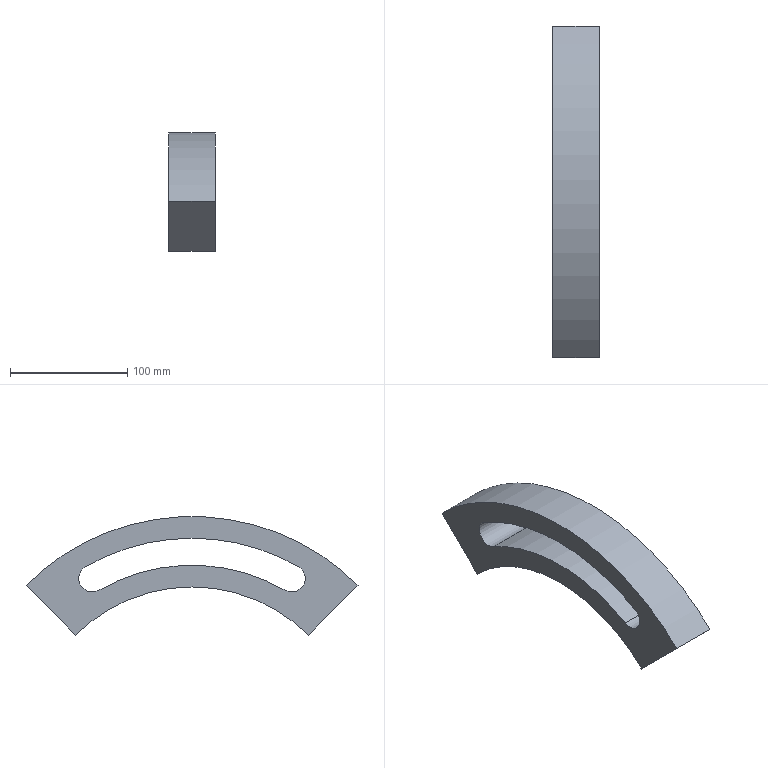Component | NX | BALANCE_BLOCK | 1 solid | 10 faces | box 40 x 282.84 x 101.01 mm | volume 460484 mm3 | cylinder 6 | plane 4 | commonest cylinder face diameters 23 x2 363 x1 280 x1 400 x1 317 x1
STEP:
#1=CARTESIAN_POINT('',(0.,0.,0.));
#2=DIRECTION('',(0.,0.,1.));
#3=DIRECTION('',(1.,0.,0.));
#4=AXIS2_PLACEMENT_3D('',#1,#2,#3);
#5=CARTESIAN_POINT('',(90.,-79.25,137.265));
#6=VERTEX_POINT('',#5);
#7=CARTESIAN_POINT('',(50.,-79.25,137.265));
#8=VERTEX_POINT('',#7);
#9=CARTESIAN_POINT('',(90.,-79.25,137.265));
#10=DIRECTION('',(-1.,0.,0.));
#11=VECTOR('',#10,1.);
#12=LINE('',#9,#11);
#13=CARTESIAN_POINT('',(90.,-85.,147.224));
#14=DIRECTION('',(-1.,0.,0.));
#15=DIRECTION('',(0.,0.,1.));
#16=AXIS2_PLACEMENT_3D('',#13,#14,#15);
#17=CYLINDRICAL_SURFACE('',#16,11.5);
#18=CARTESIAN_POINT('',(2.618,0.));
#19=DIRECTION('',(0.,1.));
#20=VECTOR('',#19,1.);
#21=LINE('',#18,#20);
#22=(GEOMETRIC_REPRESENTATION_CONTEXT(2)PARAMETRIC_REPRESENTATION_CONTEXT()REPRESENTATION_CONTEXT('',''));
#23=DEFINITIONAL_REPRESENTATION('',(#21),#22);
#24=PCURVE('',#17,#23);
#25=CARTESIAN_POINT('',(90.,0.,0.));
#26=DIRECTION('',(-1.,0.,0.));
#27=DIRECTION('',(0.,0.,1.));
#28=AXIS2_PLACEMENT_3D('',#25,#26,#27);
#29=CYLINDRICAL_SURFACE('',#28,158.5);
#30=CARTESIAN_POINT('',(-0.5236,0.));
#31=DIRECTION('',(0.,1.));
#32=VECTOR('',#31,1.);
#33=LINE('',#30,#32);
#34=(GEOMETRIC_REPRESENTATION_CONTEXT(2)PARAMETRIC_REPRESENTATION_CONTEXT()REPRESENTATION_CONTEXT('',''));
#35=DEFINITIONAL_REPRESENTATION('',(#33),#34);
#36=PCURVE('',#29,#35);
#37=SURFACE_CURVE('',#12,(#24,#36),.PCURVE_S1.);
#38=EDGE_CURVE('',#6,#8,#37,.T.);
#39=ORIENTED_EDGE('',*,*,#38,.F.);
#40=CARTESIAN_POINT('',(90.,-90.75,157.184));
#41=VERTEX_POINT('',#40);
#42=CARTESIAN_POINT('',(90.,-85.,147.224));
#43=DIRECTION('',(-1.,0.,0.));
#44=DIRECTION('',(0.,1.,0.));
#45=AXIS2_PLACEMENT_3D('',#42,#43,#44);
#46=CIRCLE('',#45,11.5);
#47=CARTESIAN_POINT('',(1.571,0.));
#48=DIRECTION('',(1.,0.));
#49=VECTOR('',#48,1.);
#50=LINE('',#47,#49);
#51=(GEOMETRIC_REPRESENTATION_CONTEXT(2)PARAMETRIC_REPRESENTATION_CONTEXT()REPRESENTATION_CONTEXT('',''));
#52=DEFINITIONAL_REPRESENTATION('',(#50),#51);
#53=PCURVE('',#17,#52);
#54=CARTESIAN_POINT('',(90.,0.,0.));
#55=DIRECTION('',(-1.,0.,0.));
#56=DIRECTION('',(0.,0.,1.));
#57=AXIS2_PLACEMENT_3D('',#54,#55,#56);
#58=PLANE('',#57);
#59=CARTESIAN_POINT('',(147.224,-85.));
#60=DIRECTION('',(0.,1.));
#61=AXIS2_PLACEMENT_2D('',#59,#60);
#62=CIRCLE('',#61,11.5);
#63=(GEOMETRIC_REPRESENTATION_CONTEXT(2)PARAMETRIC_REPRESENTATION_CONTEXT()REPRESENTATION_CONTEXT('',''));
#64=DEFINITIONAL_REPRESENTATION('',(#62),#63);
#65=PCURVE('',#58,#64);
#66=SURFACE_CURVE('',#46,(#53,#65),.PCURVE_S1.);
#67=EDGE_CURVE('',#6,#41,#66,.T.);
#68=ORIENTED_EDGE('',*,*,#67,.T.);
#69=CARTESIAN_POINT('',(50.,-90.75,157.184));
#70=VERTEX_POINT('',#69);
#71=CARTESIAN_POINT('',(90.,-90.75,157.184));
#72=DIRECTION('',(-1.,0.,0.));
#73=VECTOR('',#72,1.);
#74=LINE('',#71,#73);
#75=CARTESIAN_POINT('',(5.76,0.));
#76=DIRECTION('',(0.,1.));
#77=VECTOR('',#76,1.);
#78=LINE('',#75,#77);
#79=(GEOMETRIC_REPRESENTATION_CONTEXT(2)PARAMETRIC_REPRESENTATION_CONTEXT()REPRESENTATION_CONTEXT('',''));
#80=DEFINITIONAL_REPRESENTATION('',(#78),#79);
#81=PCURVE('',#17,#80);
#82=CARTESIAN_POINT('',(90.,0.,0.));
#83=DIRECTION('',(-1.,0.,0.));
#84=DIRECTION('',(0.,0.,1.));
#85=AXIS2_PLACEMENT_3D('',#82,#83,#84);
#86=CYLINDRICAL_SURFACE('',#85,181.5);
#87=CARTESIAN_POINT('',(5.76,0.));
#88=DIRECTION('',(0.,1.));
#89=VECTOR('',#88,1.);
#90=LINE('',#87,#89);
#91=(GEOMETRIC_REPRESENTATION_CONTEXT(2)PARAMETRIC_REPRESENTATION_CONTEXT()REPRESENTATION_CONTEXT('',''));
#92=DEFINITIONAL_REPRESENTATION('',(#90),#91);
#93=PCURVE('',#86,#92);
#94=SURFACE_CURVE('',#74,(#81,#93),.PCURVE_S1.);
#95=EDGE_CURVE('',#41,#70,#94,.T.);
#96=ORIENTED_EDGE('',*,*,#95,.T.);
#97=CARTESIAN_POINT('',(50.,-85.,147.224));
#98=DIRECTION('',(-1.,0.,0.));
#99=DIRECTION('',(0.,1.,0.));
#100=AXIS2_PLACEMENT_3D('',#97,#98,#99);
#101=CIRCLE('',#100,11.5);
#102=CARTESIAN_POINT('',(1.571,40.));
#103=DIRECTION('',(1.,0.));
#104=VECTOR('',#103,1.);
#105=LINE('',#102,#104);
#106=(GEOMETRIC_REPRESENTATION_CONTEXT(2)PARAMETRIC_REPRESENTATION_CONTEXT()REPRESENTATION_CONTEXT('',''));
#107=DEFINITIONAL_REPRESENTATION('',(#105),#106);
#108=PCURVE('',#17,#107);
#109=CARTESIAN_POINT('',(50.,0.,0.));
#110=DIRECTION('',(-1.,0.,0.));
#111=DIRECTION('',(0.,0.,1.));
#112=AXIS2_PLACEMENT_3D('',#109,#110,#111);
#113=PLANE('',#112);
#114=CARTESIAN_POINT('',(147.224,-85.));
#115=DIRECTION('',(0.,1.));
#116=AXIS2_PLACEMENT_2D('',#114,#115);
#117=CIRCLE('',#116,11.5);
#118=(GEOMETRIC_REPRESENTATION_CONTEXT(2)PARAMETRIC_REPRESENTATION_CONTEXT()REPRESENTATION_CONTEXT('',''));
#119=DEFINITIONAL_REPRESENTATION('',(#117),#118);
#120=PCURVE('',#113,#119);
#121=SURFACE_CURVE('',#101,(#108,#120),.PCURVE_S1.);
#122=EDGE_CURVE('',#8,#70,#121,.T.);
#123=ORIENTED_EDGE('',*,*,#122,.F.);
#124=EDGE_LOOP('',(#39,#68,#96,#123));
#125=FACE_BOUND('',#124,.F.);
#126=ADVANCED_FACE('',(#125),#17,.F.);
#127=ORIENTED_EDGE('',*,*,#95,.F.);
#128=CARTESIAN_POINT('',(90.,90.75,157.184));
#129=VERTEX_POINT('',#128);
#130=CARTESIAN_POINT('',(90.,0.,0.));
#131=DIRECTION('',(-1.,0.,0.));
#132=DIRECTION('',(0.,1.,0.));
#133=AXIS2_PLACEMENT_3D('',#130,#131,#132);
#134=CIRCLE('',#133,181.5);
#135=CARTESIAN_POINT('',(1.571,0.));
#136=DIRECTION('',(1.,0.));
#137=VECTOR('',#136,1.);
#138=LINE('',#135,#137);
#139=(GEOMETRIC_REPRESENTATION_CONTEXT(2)PARAMETRIC_REPRESENTATION_CONTEXT()REPRESENTATION_CONTEXT('',''));
#140=DEFINITIONAL_REPRESENTATION('',(#138),#139);
#141=PCURVE('',#86,#140);
#142=CARTESIAN_POINT('',(0.,0.));
#143=DIRECTION('',(0.,1.));
#144=AXIS2_PLACEMENT_2D('',#142,#143);
#145=CIRCLE('',#144,181.5);
#146=(GEOMETRIC_REPRESENTATION_CONTEXT(2)PARAMETRIC_REPRESENTATION_CONTEXT()REPRESENTATION_CONTEXT('',''));
#147=DEFINITIONAL_REPRESENTATION('',(#145),#146);
#148=PCURVE('',#58,#147);
#149=SURFACE_CURVE('',#134,(#141,#148),.PCURVE_S1.);
#150=EDGE_CURVE('',#41,#129,#149,.T.);
#151=ORIENTED_EDGE('',*,*,#150,.T.);
#152=CARTESIAN_POINT('',(50.,90.75,157.184));
#153=VERTEX_POINT('',#152);
#154=CARTESIAN_POINT('',(90.,90.75,157.184));
#155=DIRECTION('',(-1.,0.,0.));
#156=VECTOR('',#155,1.);
#157=LINE('',#154,#156);
#158=CARTESIAN_POINT('',(6.807,0.));
#159=DIRECTION('',(0.,1.));
#160=VECTOR('',#159,1.);
#161=LINE('',#158,#160);
#162=(GEOMETRIC_REPRESENTATION_CONTEXT(2)PARAMETRIC_REPRESENTATION_CONTEXT()REPRESENTATION_CONTEXT('',''));
#163=DEFINITIONAL_REPRESENTATION('',(#161),#162);
#164=PCURVE('',#86,#163);
#165=CARTESIAN_POINT('',(90.,85.,147.224));
#166=DIRECTION('',(-1.,0.,0.));
#167=DIRECTION('',(0.,0.,1.));
#168=AXIS2_PLACEMENT_3D('',#165,#166,#167);
#169=CYLINDRICAL_SURFACE('',#168,11.5);
#170=CARTESIAN_POINT('',(0.5236,0.));
#171=DIRECTION('',(0.,1.));
#172=VECTOR('',#171,1.);
#173=LINE('',#170,#172);
#174=(GEOMETRIC_REPRESENTATION_CONTEXT(2)PARAMETRIC_REPRESENTATION_CONTEXT()REPRESENTATION_CONTEXT('',''));
#175=DEFINITIONAL_REPRESENTATION('',(#173),#174);
#176=PCURVE('',#169,#175);
#177=SURFACE_CURVE('',#157,(#164,#176),.PCURVE_S1.);
#178=EDGE_CURVE('',#129,#153,#177,.T.);
#179=ORIENTED_EDGE('',*,*,#178,.T.);
#180=CARTESIAN_POINT('',(50.,0.,0.));
#181=DIRECTION('',(-1.,0.,0.));
#182=DIRECTION('',(0.,1.,0.));
#183=AXIS2_PLACEMENT_3D('',#180,#181,#182);
#184=CIRCLE('',#183,181.5);
#185=CARTESIAN_POINT('',(1.571,40.));
#186=DIRECTION('',(1.,0.));
#187=VECTOR('',#186,1.);
#188=LINE('',#185,#187);
#189=(GEOMETRIC_REPRESENTATION_CONTEXT(2)PARAMETRIC_REPRESENTATION_CONTEXT()REPRESENTATION_CONTEXT('',''));
#190=DEFINITIONAL_REPRESENTATION('',(#188),#189);
#191=PCURVE('',#86,#190);
#192=CARTESIAN_POINT('',(0.,0.));
#193=DIRECTION('',(0.,1.));
#194=AXIS2_PLACEMENT_2D('',#192,#193);
#195=CIRCLE('',#194,181.5);
#196=(GEOMETRIC_REPRESENTATION_CONTEXT(2)PARAMETRIC_REPRESENTATION_CONTEXT()REPRESENTATION_CONTEXT('',''));
#197=DEFINITIONAL_REPRESENTATION('',(#195),#196);
#198=PCURVE('',#113,#197);
#199=SURFACE_CURVE('',#184,(#191,#198),.PCURVE_S1.);
#200=EDGE_CURVE('',#70,#153,#199,.T.);
#201=ORIENTED_EDGE('',*,*,#200,.F.);
#202=EDGE_LOOP('',(#127,#151,#179,#201));
#203=FACE_BOUND('',#202,.F.);
#204=ADVANCED_FACE('',(#203),#86,.F.);
#205=ORIENTED_EDGE('',*,*,#178,.F.);
#206=CARTESIAN_POINT('',(90.,79.25,137.265));
#207=VERTEX_POINT('',#206);
#208=CARTESIAN_POINT('',(90.,85.,147.224));
#209=DIRECTION('',(-1.,0.,0.));
#210=DIRECTION('',(0.,1.,0.));
#211=AXIS2_PLACEMENT_3D('',#208,#209,#210);
#212=CIRCLE('',#211,11.5);
#213=CARTESIAN_POINT('',(-4.712,0.));
#214=DIRECTION('',(1.,0.));
#215=VECTOR('',#214,1.);
#216=LINE('',#213,#215);
#217=(GEOMETRIC_REPRESENTATION_CONTEXT(2)PARAMETRIC_REPRESENTATION_CONTEXT()REPRESENTATION_CONTEXT('',''));
#218=DEFINITIONAL_REPRESENTATION('',(#216),#217);
#219=PCURVE('',#169,#218);
#220=CARTESIAN_POINT('',(147.224,85.));
#221=DIRECTION('',(0.,1.));
#222=AXIS2_PLACEMENT_2D('',#220,#221);
#223=CIRCLE('',#222,11.5);
#224=(GEOMETRIC_REPRESENTATION_CONTEXT(2)PARAMETRIC_REPRESENTATION_CONTEXT()REPRESENTATION_CONTEXT('',''));
#225=DEFINITIONAL_REPRESENTATION('',(#223),#224);
#226=PCURVE('',#58,#225);
#227=SURFACE_CURVE('',#212,(#219,#226),.PCURVE_S1.);
#228=EDGE_CURVE('',#129,#207,#227,.T.);
#229=ORIENTED_EDGE('',*,*,#228,.T.);
#230=CARTESIAN_POINT('',(50.,79.25,137.265));
#231=VERTEX_POINT('',#230);
#232=CARTESIAN_POINT('',(90.,79.25,137.265));
#233=DIRECTION('',(-1.,0.,0.));
#234=VECTOR('',#233,1.);
#235=LINE('',#232,#234);
#236=CARTESIAN_POINT('',(3.665,0.));
#237=DIRECTION('',(0.,1.));
#238=VECTOR('',#237,1.);
#239=LINE('',#236,#238);
#240=(GEOMETRIC_REPRESENTATION_CONTEXT(2)PARAMETRIC_REPRESENTATION_CONTEXT()REPRESENTATION_CONTEXT('',''));
#241=DEFINITIONAL_REPRESENTATION('',(#239),#240);
#242=PCURVE('',#169,#241);
#243=CARTESIAN_POINT('',(0.5236,0.));
#244=DIRECTION('',(0.,1.));
#245=VECTOR('',#244,1.);
#246=LINE('',#243,#245);
#247=(GEOMETRIC_REPRESENTATION_CONTEXT(2)PARAMETRIC_REPRESENTATION_CONTEXT()REPRESENTATION_CONTEXT('',''));
#248=DEFINITIONAL_REPRESENTATION('',(#246),#247);
#249=PCURVE('',#29,#248);
#250=SURFACE_CURVE('',#235,(#242,#249),.PCURVE_S1.);
#251=EDGE_CURVE('',#207,#231,#250,.T.);
#252=ORIENTED_EDGE('',*,*,#251,.T.);
#253=CARTESIAN_POINT('',(50.,85.,147.224));
#254=DIRECTION('',(-1.,0.,0.));
#255=DIRECTION('',(0.,1.,0.));
#256=AXIS2_PLACEMENT_3D('',#253,#254,#255);
#257=CIRCLE('',#256,11.5);
#258=CARTESIAN_POINT('',(-4.712,40.));
#259=DIRECTION('',(1.,0.));
#260=VECTOR('',#259,1.);
#261=LINE('',#258,#260);
#262=(GEOMETRIC_REPRESENTATION_CONTEXT(2)PARAMETRIC_REPRESENTATION_CONTEXT()REPRESENTATION_CONTEXT('',''));
#263=DEFINITIONAL_REPRESENTATION('',(#261),#262);
#264=PCURVE('',#169,#263);
#265=CARTESIAN_POINT('',(147.224,85.));
#266=DIRECTION('',(0.,1.));
#267=AXIS2_PLACEMENT_2D('',#265,#266);
#268=CIRCLE('',#267,11.5);
#269=(GEOMETRIC_REPRESENTATION_CONTEXT(2)PARAMETRIC_REPRESENTATION_CONTEXT()REPRESENTATION_CONTEXT('',''));
#270=DEFINITIONAL_REPRESENTATION('',(#268),#269);
#271=PCURVE('',#113,#270);
#272=SURFACE_CURVE('',#257,(#264,#271),.PCURVE_S1.);
#273=EDGE_CURVE('',#153,#231,#272,.T.);
#274=ORIENTED_EDGE('',*,*,#273,.F.);
#275=EDGE_LOOP('',(#205,#229,#252,#274));
#276=FACE_BOUND('',#275,.F.);
#277=ADVANCED_FACE('',(#276),#169,.F.);
#278=CARTESIAN_POINT('',(50.,-141.421,141.421));
#279=VERTEX_POINT('',#278);
#280=CARTESIAN_POINT('',(50.,-98.995,98.995));
#281=VERTEX_POINT('',#280);
#282=CARTESIAN_POINT('',(50.,-141.421,141.421));
#283=DIRECTION('',(0.,0.7071,-0.7071));
#284=VECTOR('',#283,1.);
#285=LINE('',#282,#284);
#286=CARTESIAN_POINT('',(90.,-141.421,141.421));
#287=DIRECTION('',(0.,0.7071,0.7071));
#288=DIRECTION('',(0.,-0.7071,0.7071));
#289=AXIS2_PLACEMENT_3D('',#286,#287,#288);
#290=PLANE('',#289);
#291=CARTESIAN_POINT('',(0.,-40.));
#292=DIRECTION('',(-1.,0.));
#293=VECTOR('',#292,1.);
#294=LINE('',#291,#293);
#295=(GEOMETRIC_REPRESENTATION_CONTEXT(2)PARAMETRIC_REPRESENTATION_CONTEXT()REPRESENTATION_CONTEXT('',''));
#296=DEFINITIONAL_REPRESENTATION('',(#294),#295);
#297=PCURVE('',#290,#296);
#298=CARTESIAN_POINT('',(141.421,-141.421));
#299=DIRECTION('',(-0.7071,0.7071));
#300=VECTOR('',#299,1.);
#301=LINE('',#298,#300);
#302=(GEOMETRIC_REPRESENTATION_CONTEXT(2)PARAMETRIC_REPRESENTATION_CONTEXT()REPRESENTATION_CONTEXT('',''));
#303=DEFINITIONAL_REPRESENTATION('',(#301),#302);
#304=PCURVE('',#113,#303);
#305=SURFACE_CURVE('',#285,(#297,#304),.PCURVE_S1.);
#306=EDGE_CURVE('',#279,#281,#305,.T.);
#307=ORIENTED_EDGE('',*,*,#306,.T.);
#308=CARTESIAN_POINT('',(90.,-98.995,98.995));
#309=VERTEX_POINT('',#308);
#310=CARTESIAN_POINT('',(90.,-98.995,98.995));
#311=DIRECTION('',(-1.,0.,0.));
#312=VECTOR('',#311,1.);
#313=LINE('',#310,#312);
#314=CARTESIAN_POINT('',(-60.,0.));
#315=DIRECTION('',(0.,-1.));
#316=VECTOR('',#315,1.);
#317=LINE('',#314,#316);
#318=(GEOMETRIC_REPRESENTATION_CONTEXT(2)PARAMETRIC_REPRESENTATION_CONTEXT()REPRESENTATION_CONTEXT('',''));
#319=DEFINITIONAL_REPRESENTATION('',(#317),#318);
#320=PCURVE('',#290,#319);
#321=CARTESIAN_POINT('',(90.,0.,0.));
#322=DIRECTION('',(-1.,0.,0.));
#323=DIRECTION('',(0.,0.,1.));
#324=AXIS2_PLACEMENT_3D('',#321,#322,#323);
#325=CYLINDRICAL_SURFACE('',#324,140.);
#326=CARTESIAN_POINT('',(5.498,0.));
#327=DIRECTION('',(0.,1.));
#328=VECTOR('',#327,1.);
#329=LINE('',#326,#328);
#330=(GEOMETRIC_REPRESENTATION_CONTEXT(2)PARAMETRIC_REPRESENTATION_CONTEXT()REPRESENTATION_CONTEXT('',''));
#331=DEFINITIONAL_REPRESENTATION('',(#329),#330);
#332=PCURVE('',#325,#331);
#333=SURFACE_CURVE('',#313,(#320,#332),.PCURVE_S1.);
#334=EDGE_CURVE('',#309,#281,#333,.T.);
#335=ORIENTED_EDGE('',*,*,#334,.F.);
#336=CARTESIAN_POINT('',(90.,-141.421,141.421));
#337=VERTEX_POINT('',#336);
#338=CARTESIAN_POINT('',(90.,-141.421,141.421));
#339=DIRECTION('',(0.,0.7071,-0.7071));
#340=VECTOR('',#339,1.);
#341=LINE('',#338,#340);
#342=CARTESIAN_POINT('',(0.,0.));
#343=DIRECTION('',(-1.,0.));
#344=VECTOR('',#343,1.);
#345=LINE('',#342,#344);
#346=(GEOMETRIC_REPRESENTATION_CONTEXT(2)PARAMETRIC_REPRESENTATION_CONTEXT()REPRESENTATION_CONTEXT('',''));
#347=DEFINITIONAL_REPRESENTATION('',(#345),#346);
#348=PCURVE('',#290,#347);
#349=CARTESIAN_POINT('',(141.421,-141.421));
#350=DIRECTION('',(-0.7071,0.7071));
#351=VECTOR('',#350,1.);
#352=LINE('',#349,#351);
#353=(GEOMETRIC_REPRESENTATION_CONTEXT(2)PARAMETRIC_REPRESENTATION_CONTEXT()REPRESENTATION_CONTEXT('',''));
#354=DEFINITIONAL_REPRESENTATION('',(#352),#353);
#355=PCURVE('',#58,#354);
#356=SURFACE_CURVE('',#341,(#348,#355),.PCURVE_S1.);
#357=EDGE_CURVE('',#337,#309,#356,.T.);
#358=ORIENTED_EDGE('',*,*,#357,.F.);
#359=CARTESIAN_POINT('',(90.,-141.421,141.421));
#360=DIRECTION('',(-1.,0.,0.));
#361=VECTOR('',#360,1.);
#362=LINE('',#359,#361);
#363=CARTESIAN_POINT('',(0.,0.));
#364=DIRECTION('',(0.,-1.));
#365=VECTOR('',#364,1.);
#366=LINE('',#363,#365);
#367=(GEOMETRIC_REPRESENTATION_CONTEXT(2)PARAMETRIC_REPRESENTATION_CONTEXT()REPRESENTATION_CONTEXT('',''));
#368=DEFINITIONAL_REPRESENTATION('',(#366),#367);
#369=PCURVE('',#290,#368);
#370=CARTESIAN_POINT('',(90.,0.,0.));
#371=DIRECTION('',(-1.,0.,0.));
#372=DIRECTION('',(0.,0.,1.));
#373=AXIS2_PLACEMENT_3D('',#370,#371,#372);
#374=CYLINDRICAL_SURFACE('',#373,200.);
#375=CARTESIAN_POINT('',(-0.7854,0.));
#376=DIRECTION('',(0.,1.));
#377=VECTOR('',#376,1.);
#378=LINE('',#375,#377);
#379=(GEOMETRIC_REPRESENTATION_CONTEXT(2)PARAMETRIC_REPRESENTATION_CONTEXT()REPRESENTATION_CONTEXT('',''));
#380=DEFINITIONAL_REPRESENTATION('',(#378),#379);
#381=PCURVE('',#374,#380);
#382=SURFACE_CURVE('',#362,(#369,#381),.PCURVE_S1.);
#383=EDGE_CURVE('',#337,#279,#382,.T.);
#384=ORIENTED_EDGE('',*,*,#383,.T.);
#385=EDGE_LOOP('',(#307,#335,#358,#384));
#386=FACE_BOUND('',#385,.T.);
#387=ADVANCED_FACE('',(#386),#290,.F.);
#388=ORIENTED_EDGE('',*,*,#334,.F.);
#389=CARTESIAN_POINT('',(90.,98.995,98.995));
#390=VERTEX_POINT('',#389);
#391=CARTESIAN_POINT('',(90.,0.,0.));
#392=DIRECTION('',(-1.,0.,0.));
#393=DIRECTION('',(0.,1.,0.));
#394=AXIS2_PLACEMENT_3D('',#391,#392,#393);
#395=CIRCLE('',#394,140.);
#396=CARTESIAN_POINT('',(1.571,0.));
#397=DIRECTION('',(1.,0.));
#398=VECTOR('',#397,1.);
#399=LINE('',#396,#398);
#400=(GEOMETRIC_REPRESENTATION_CONTEXT(2)PARAMETRIC_REPRESENTATION_CONTEXT()REPRESENTATION_CONTEXT('',''));
#401=DEFINITIONAL_REPRESENTATION('',(#399),#400);
#402=PCURVE('',#325,#401);
#403=CARTESIAN_POINT('',(0.,0.));
#404=DIRECTION('',(0.,1.));
#405=AXIS2_PLACEMENT_2D('',#403,#404);
#406=CIRCLE('',#405,140.);
#407=(GEOMETRIC_REPRESENTATION_CONTEXT(2)PARAMETRIC_REPRESENTATION_CONTEXT()REPRESENTATION_CONTEXT('',''));
#408=DEFINITIONAL_REPRESENTATION('',(#406),#407);
#409=PCURVE('',#58,#408);
#410=SURFACE_CURVE('',#395,(#402,#409),.PCURVE_S1.);
#411=EDGE_CURVE('',#309,#390,#410,.T.);
#412=ORIENTED_EDGE('',*,*,#411,.T.);
#413=CARTESIAN_POINT('',(50.,98.995,98.995));
#414=VERTEX_POINT('',#413);
#415=CARTESIAN_POINT('',(90.,98.995,98.995));
#416=DIRECTION('',(-1.,0.,0.));
#417=VECTOR('',#416,1.);
#418=LINE('',#415,#417);
#419=CARTESIAN_POINT('',(7.069,0.));
#420=DIRECTION('',(0.,1.));
#421=VECTOR('',#420,1.);
#422=LINE('',#419,#421);
#423=(GEOMETRIC_REPRESENTATION_CONTEXT(2)PARAMETRIC_REPRESENTATION_CONTEXT()REPRESENTATION_CONTEXT('',''));
#424=DEFINITIONAL_REPRESENTATION('',(#422),#423);
#425=PCURVE('',#325,#424);
#426=CARTESIAN_POINT('',(90.,98.995,98.995));
#427=DIRECTION('',(0.,-0.7071,0.7071));
#428=DIRECTION('',(0.,-0.7071,-0.7071));
#429=AXIS2_PLACEMENT_3D('',#426,#427,#428);
#430=PLANE('',#429);
#431=CARTESIAN_POINT('',(0.,0.));
#432=DIRECTION('',(0.,-1.));
#433=VECTOR('',#432,1.);
#434=LINE('',#431,#433);
#435=(GEOMETRIC_REPRESENTATION_CONTEXT(2)PARAMETRIC_REPRESENTATION_CONTEXT()REPRESENTATION_CONTEXT('',''));
#436=DEFINITIONAL_REPRESENTATION('',(#434),#435);
#437=PCURVE('',#430,#436);
#438=SURFACE_CURVE('',#418,(#425,#437),.PCURVE_S1.);
#439=EDGE_CURVE('',#390,#414,#438,.T.);
#440=ORIENTED_EDGE('',*,*,#439,.T.);
#441=CARTESIAN_POINT('',(50.,0.,0.));
#442=DIRECTION('',(-1.,0.,0.));
#443=DIRECTION('',(0.,1.,0.));
#444=AXIS2_PLACEMENT_3D('',#441,#442,#443);
#445=CIRCLE('',#444,140.);
#446=CARTESIAN_POINT('',(1.571,40.));
#447=DIRECTION('',(1.,0.));
#448=VECTOR('',#447,1.);
#449=LINE('',#446,#448);
#450=(GEOMETRIC_REPRESENTATION_CONTEXT(2)PARAMETRIC_REPRESENTATION_CONTEXT()REPRESENTATION_CONTEXT('',''));
#451=DEFINITIONAL_REPRESENTATION('',(#449),#450);
#452=PCURVE('',#325,#451);
#453=CARTESIAN_POINT('',(0.,0.));
#454=DIRECTION('',(0.,1.));
#455=AXIS2_PLACEMENT_2D('',#453,#454);
#456=CIRCLE('',#455,140.);
#457=(GEOMETRIC_REPRESENTATION_CONTEXT(2)PARAMETRIC_REPRESENTATION_CONTEXT()REPRESENTATION_CONTEXT('',''));
#458=DEFINITIONAL_REPRESENTATION('',(#456),#457);
#459=PCURVE('',#113,#458);
#460=SURFACE_CURVE('',#445,(#452,#459),.PCURVE_S1.);
#461=EDGE_CURVE('',#281,#414,#460,.T.);
#462=ORIENTED_EDGE('',*,*,#461,.F.);
#463=EDGE_LOOP('',(#388,#412,#440,#462));
#464=FACE_BOUND('',#463,.F.);
#465=ADVANCED_FACE('',(#464),#325,.F.);
#466=CARTESIAN_POINT('',(50.,141.421,141.421));
#467=VERTEX_POINT('',#466);
#468=CARTESIAN_POINT('',(50.,98.995,98.995));
#469=DIRECTION('',(0.,0.7071,0.7071));
#470=VECTOR('',#469,1.);
#471=LINE('',#468,#470);
#472=CARTESIAN_POINT('',(0.,-40.));
#473=DIRECTION('',(-1.,0.));
#474=VECTOR('',#473,1.);
#475=LINE('',#472,#474);
#476=(GEOMETRIC_REPRESENTATION_CONTEXT(2)PARAMETRIC_REPRESENTATION_CONTEXT()REPRESENTATION_CONTEXT('',''));
#477=DEFINITIONAL_REPRESENTATION('',(#475),#476);
#478=PCURVE('',#430,#477);
#479=CARTESIAN_POINT('',(98.995,98.995));
#480=DIRECTION('',(0.7071,0.7071));
#481=VECTOR('',#480,1.);
#482=LINE('',#479,#481);
#483=(GEOMETRIC_REPRESENTATION_CONTEXT(2)PARAMETRIC_REPRESENTATION_CONTEXT()REPRESENTATION_CONTEXT('',''));
#484=DEFINITIONAL_REPRESENTATION('',(#482),#483);
#485=PCURVE('',#113,#484);
#486=SURFACE_CURVE('',#471,(#478,#485),.PCURVE_S1.);
#487=EDGE_CURVE('',#414,#467,#486,.T.);
#488=ORIENTED_EDGE('',*,*,#487,.T.);
#489=CARTESIAN_POINT('',(90.,141.421,141.421));
#490=VERTEX_POINT('',#489);
#491=CARTESIAN_POINT('',(90.,141.421,141.421));
#492=DIRECTION('',(-1.,0.,0.));
#493=VECTOR('',#492,1.);
#494=LINE('',#491,#493);
#495=CARTESIAN_POINT('',(-60.,0.));
#496=DIRECTION('',(0.,-1.));
#497=VECTOR('',#496,1.);
#498=LINE('',#495,#497);
#499=(GEOMETRIC_REPRESENTATION_CONTEXT(2)PARAMETRIC_REPRESENTATION_CONTEXT()REPRESENTATION_CONTEXT('',''));
#500=DEFINITIONAL_REPRESENTATION('',(#498),#499);
#501=PCURVE('',#430,#500);
#502=CARTESIAN_POINT('',(0.7854,0.));
#503=DIRECTION('',(0.,1.));
#504=VECTOR('',#503,1.);
#505=LINE('',#502,#504);
#506=(GEOMETRIC_REPRESENTATION_CONTEXT(2)PARAMETRIC_REPRESENTATION_CONTEXT()REPRESENTATION_CONTEXT('',''));
#507=DEFINITIONAL_REPRESENTATION('',(#505),#506);
#508=PCURVE('',#374,#507);
#509=SURFACE_CURVE('',#494,(#501,#508),.PCURVE_S1.);
#510=EDGE_CURVE('',#490,#467,#509,.T.);
#511=ORIENTED_EDGE('',*,*,#510,.F.);
#512=CARTESIAN_POINT('',(90.,98.995,98.995));
#513=DIRECTION('',(0.,0.7071,0.7071));
#514=VECTOR('',#513,1.);
#515=LINE('',#512,#514);
#516=CARTESIAN_POINT('',(0.,0.));
#517=DIRECTION('',(-1.,0.));
#518=VECTOR('',#517,1.);
#519=LINE('',#516,#518);
#520=(GEOMETRIC_REPRESENTATION_CONTEXT(2)PARAMETRIC_REPRESENTATION_CONTEXT()REPRESENTATION_CONTEXT('',''));
#521=DEFINITIONAL_REPRESENTATION('',(#519),#520);
#522=PCURVE('',#430,#521);
#523=CARTESIAN_POINT('',(98.995,98.995));
#524=DIRECTION('',(0.7071,0.7071));
#525=VECTOR('',#524,1.);
#526=LINE('',#523,#525);
#527=(GEOMETRIC_REPRESENTATION_CONTEXT(2)PARAMETRIC_REPRESENTATION_CONTEXT()REPRESENTATION_CONTEXT('',''));
#528=DEFINITIONAL_REPRESENTATION('',(#526),#527);
#529=PCURVE('',#58,#528);
#530=SURFACE_CURVE('',#515,(#522,#529),.PCURVE_S1.);
#531=EDGE_CURVE('',#390,#490,#530,.T.);
#532=ORIENTED_EDGE('',*,*,#531,.F.);
#533=ORIENTED_EDGE('',*,*,#439,.T.);
#534=EDGE_LOOP('',(#488,#511,#532,#533));
#535=FACE_BOUND('',#534,.T.);
#536=ADVANCED_FACE('',(#535),#430,.F.);
#537=CARTESIAN_POINT('',(50.,0.,0.));
#538=DIRECTION('',(1.,0.,0.));
#539=DIRECTION('',(0.,1.,-0.));
#540=AXIS2_PLACEMENT_3D('',#537,#538,#539);
#541=CIRCLE('',#540,200.);
#542=CARTESIAN_POINT('',(1.571,40.));
#543=DIRECTION('',(-1.,0.));
#544=VECTOR('',#543,1.);
#545=LINE('',#542,#544);
#546=(GEOMETRIC_REPRESENTATION_CONTEXT(2)PARAMETRIC_REPRESENTATION_CONTEXT()REPRESENTATION_CONTEXT('',''));
#547=DEFINITIONAL_REPRESENTATION('',(#545),#546);
#548=PCURVE('',#374,#547);
#549=CARTESIAN_POINT('',(-0.,200.));
#550=CARTESIAN_POINT('',(346.41,200.));
#551=CARTESIAN_POINT('',(173.205,-100.));
#552=CARTESIAN_POINT('',(0.,-400.));
#553=CARTESIAN_POINT('',(-173.205,-100.));
#554=CARTESIAN_POINT('',(-346.41,200.));
#555=CARTESIAN_POINT('',(-0.,200.));
#556=(BOUNDED_CURVE()B_SPLINE_CURVE(2,(#549,#550,#551,#552,#553,#554,#555),.UNSPECIFIED.,.T.,.F.)B_SPLINE_CURVE_WITH_KNOTS((1,2,2,2,2,1),(-2.094,0.,2.094,4.189,6.283,8.378),.UNSPECIFIED.)CURVE()GEOMETRIC_REPRESENTATION_ITEM()RATIONAL_B_SPLINE_CURVE((1.,0.5,1.,0.5,1.,0.5,1.))REPRESENTATION_ITEM(''));
#557=(GEOMETRIC_REPRESENTATION_CONTEXT(2)PARAMETRIC_REPRESENTATION_CONTEXT()REPRESENTATION_CONTEXT('',''));
#558=DEFINITIONAL_REPRESENTATION('',(#556),#557);
#559=PCURVE('',#113,#558);
#560=SURFACE_CURVE('',#541,(#548,#559),.PCURVE_S1.);
#561=EDGE_CURVE('',#467,#279,#560,.T.);
#562=ORIENTED_EDGE('',*,*,#561,.T.);
#563=ORIENTED_EDGE('',*,*,#383,.F.);
#564=CARTESIAN_POINT('',(90.,0.,0.));
#565=DIRECTION('',(1.,0.,0.));
#566=DIRECTION('',(0.,1.,-0.));
#567=AXIS2_PLACEMENT_3D('',#564,#565,#566);
#568=CIRCLE('',#567,200.);
#569=CARTESIAN_POINT('',(1.571,0.));
#570=DIRECTION('',(-1.,0.));
#571=VECTOR('',#570,1.);
#572=LINE('',#569,#571);
#573=(GEOMETRIC_REPRESENTATION_CONTEXT(2)PARAMETRIC_REPRESENTATION_CONTEXT()REPRESENTATION_CONTEXT('',''));
#574=DEFINITIONAL_REPRESENTATION('',(#572),#573);
#575=PCURVE('',#374,#574);
#576=CARTESIAN_POINT('',(-0.,200.));
#577=CARTESIAN_POINT('',(346.41,200.));
#578=CARTESIAN_POINT('',(173.205,-100.));
#579=CARTESIAN_POINT('',(0.,-400.));
#580=CARTESIAN_POINT('',(-173.205,-100.));
#581=CARTESIAN_POINT('',(-346.41,200.));
#582=CARTESIAN_POINT('',(-0.,200.));
#583=(BOUNDED_CURVE()B_SPLINE_CURVE(2,(#576,#577,#578,#579,#580,#581,#582),.UNSPECIFIED.,.T.,.F.)B_SPLINE_CURVE_WITH_KNOTS((1,2,2,2,2,1),(-2.094,0.,2.094,4.189,6.283,8.378),.UNSPECIFIED.)CURVE()GEOMETRIC_REPRESENTATION_ITEM()RATIONAL_B_SPLINE_CURVE((1.,0.5,1.,0.5,1.,0.5,1.))REPRESENTATION_ITEM(''));
#584=(GEOMETRIC_REPRESENTATION_CONTEXT(2)PARAMETRIC_REPRESENTATION_CONTEXT()REPRESENTATION_CONTEXT('',''));
#585=DEFINITIONAL_REPRESENTATION('',(#583),#584);
#586=PCURVE('',#58,#585);
#587=SURFACE_CURVE('',#568,(#575,#586),.PCURVE_S1.);
#588=EDGE_CURVE('',#490,#337,#587,.T.);
#589=ORIENTED_EDGE('',*,*,#588,.F.);
#590=ORIENTED_EDGE('',*,*,#510,.T.);
#591=EDGE_LOOP('',(#562,#563,#589,#590));
#592=FACE_BOUND('',#591,.T.);
#593=ADVANCED_FACE('',(#592),#374,.T.);
#594=CARTESIAN_POINT('',(50.,0.,0.));
#595=DIRECTION('',(1.,0.,0.));
#596=DIRECTION('',(0.,1.,-0.));
#597=AXIS2_PLACEMENT_3D('',#594,#595,#596);
#598=CIRCLE('',#597,158.5);
#599=CARTESIAN_POINT('',(1.571,40.));
#600=DIRECTION('',(-1.,0.));
#601=VECTOR('',#600,1.);
#602=LINE('',#599,#601);
#603=(GEOMETRIC_REPRESENTATION_CONTEXT(2)PARAMETRIC_REPRESENTATION_CONTEXT()REPRESENTATION_CONTEXT('',''));
#604=DEFINITIONAL_REPRESENTATION('',(#602),#603);
#605=PCURVE('',#29,#604);
#606=CARTESIAN_POINT('',(-0.,158.5));
#607=CARTESIAN_POINT('',(274.53,158.5));
#608=CARTESIAN_POINT('',(137.265,-79.25));
#609=CARTESIAN_POINT('',(0.,-317.));
#610=CARTESIAN_POINT('',(-137.265,-79.25));
#611=CARTESIAN_POINT('',(-274.53,158.5));
#612=CARTESIAN_POINT('',(-0.,158.5));
#613=(BOUNDED_CURVE()B_SPLINE_CURVE(2,(#606,#607,#608,#609,#610,#611,#612),.UNSPECIFIED.,.T.,.F.)B_SPLINE_CURVE_WITH_KNOTS((1,2,2,2,2,1),(-2.094,0.,2.094,4.189,6.283,8.378),.UNSPECIFIED.)CURVE()GEOMETRIC_REPRESENTATION_ITEM()RATIONAL_B_SPLINE_CURVE((1.,0.5,1.,0.5,1.,0.5,1.))REPRESENTATION_ITEM(''));
#614=(GEOMETRIC_REPRESENTATION_CONTEXT(2)PARAMETRIC_REPRESENTATION_CONTEXT()REPRESENTATION_CONTEXT('',''));
#615=DEFINITIONAL_REPRESENTATION('',(#613),#614);
#616=PCURVE('',#113,#615);
#617=SURFACE_CURVE('',#598,(#605,#616),.PCURVE_S1.);
#618=EDGE_CURVE('',#231,#8,#617,.T.);
#619=ORIENTED_EDGE('',*,*,#618,.T.);
#620=ORIENTED_EDGE('',*,*,#38,.F.);
#621=CARTESIAN_POINT('',(90.,0.,0.));
#622=DIRECTION('',(1.,0.,0.));
#623=DIRECTION('',(0.,1.,-0.));
#624=AXIS2_PLACEMENT_3D('',#621,#622,#623);
#625=CIRCLE('',#624,158.5);
#626=CARTESIAN_POINT('',(1.571,0.));
#627=DIRECTION('',(-1.,0.));
#628=VECTOR('',#627,1.);
#629=LINE('',#626,#628);
#630=(GEOMETRIC_REPRESENTATION_CONTEXT(2)PARAMETRIC_REPRESENTATION_CONTEXT()REPRESENTATION_CONTEXT('',''));
#631=DEFINITIONAL_REPRESENTATION('',(#629),#630);
#632=PCURVE('',#29,#631);
#633=CARTESIAN_POINT('',(-0.,158.5));
#634=CARTESIAN_POINT('',(274.53,158.5));
#635=CARTESIAN_POINT('',(137.265,-79.25));
#636=CARTESIAN_POINT('',(0.,-317.));
#637=CARTESIAN_POINT('',(-137.265,-79.25));
#638=CARTESIAN_POINT('',(-274.53,158.5));
#639=CARTESIAN_POINT('',(-0.,158.5));
#640=(BOUNDED_CURVE()B_SPLINE_CURVE(2,(#633,#634,#635,#636,#637,#638,#639),.UNSPECIFIED.,.T.,.F.)B_SPLINE_CURVE_WITH_KNOTS((1,2,2,2,2,1),(-2.094,0.,2.094,4.189,6.283,8.378),.UNSPECIFIED.)CURVE()GEOMETRIC_REPRESENTATION_ITEM()RATIONAL_B_SPLINE_CURVE((1.,0.5,1.,0.5,1.,0.5,1.))REPRESENTATION_ITEM(''));
#641=(GEOMETRIC_REPRESENTATION_CONTEXT(2)PARAMETRIC_REPRESENTATION_CONTEXT()REPRESENTATION_CONTEXT('',''));
#642=DEFINITIONAL_REPRESENTATION('',(#640),#641);
#643=PCURVE('',#58,#642);
#644=SURFACE_CURVE('',#625,(#632,#643),.PCURVE_S1.);
#645=EDGE_CURVE('',#207,#6,#644,.T.);
#646=ORIENTED_EDGE('',*,*,#645,.F.);
#647=ORIENTED_EDGE('',*,*,#251,.T.);
#648=EDGE_LOOP('',(#619,#620,#646,#647));
#649=FACE_BOUND('',#648,.T.);
#650=ADVANCED_FACE('',(#649),#29,.T.);
#651=ORIENTED_EDGE('',*,*,#357,.T.);
#652=ORIENTED_EDGE('',*,*,#411,.T.);
#653=ORIENTED_EDGE('',*,*,#531,.T.);
#654=ORIENTED_EDGE('',*,*,#588,.T.);
#655=EDGE_LOOP('',(#651,#652,#653,#654));
#656=FACE_BOUND('',#655,.T.);
#657=ORIENTED_EDGE('',*,*,#67,.T.);
#658=ORIENTED_EDGE('',*,*,#150,.T.);
#659=ORIENTED_EDGE('',*,*,#228,.T.);
#660=ORIENTED_EDGE('',*,*,#645,.T.);
#661=EDGE_LOOP('',(#657,#658,#659,#660));
#662=FACE_BOUND('',#661,.T.);
#663=ADVANCED_FACE('',(#656,#662),#58,.F.);
#664=ORIENTED_EDGE('',*,*,#306,.F.);
#665=ORIENTED_EDGE('',*,*,#561,.F.);
#666=ORIENTED_EDGE('',*,*,#487,.F.);
#667=ORIENTED_EDGE('',*,*,#461,.F.);
#668=EDGE_LOOP('',(#664,#665,#666,#667));
#669=FACE_BOUND('',#668,.T.);
#670=ORIENTED_EDGE('',*,*,#122,.F.);
#671=ORIENTED_EDGE('',*,*,#618,.F.);
#672=ORIENTED_EDGE('',*,*,#273,.F.);
#673=ORIENTED_EDGE('',*,*,#200,.F.);
#674=EDGE_LOOP('',(#670,#671,#672,#673));
#675=FACE_BOUND('',#674,.T.);
#676=ADVANCED_FACE('',(#669,#675),#113,.T.);
#677=CLOSED_SHELL('',(#126,#204,#277,#387,#465,#536,#593,#650,#663,#676));
#678=MANIFOLD_SOLID_BREP('',#677);
#679=(LENGTH_UNIT()NAMED_UNIT(*)SI_UNIT(.MILLI.,.METRE.));
#680=UNCERTAINTY_MEASURE_WITH_UNIT(LENGTH_MEASURE(0.0000001),#679,'','');
#681=(NAMED_UNIT(*)PLANE_ANGLE_UNIT()SI_UNIT($,.RADIAN.));
#682=(NAMED_UNIT(*)SI_UNIT($,.STERADIAN.)SOLID_ANGLE_UNIT());
#683=(GEOMETRIC_REPRESENTATION_CONTEXT(3)GLOBAL_UNCERTAINTY_ASSIGNED_CONTEXT((#680))GLOBAL_UNIT_ASSIGNED_CONTEXT((#679,#681,#682))REPRESENTATION_CONTEXT('',''));
#684=ADVANCED_BREP_SHAPE_REPRESENTATION('',(#4,#678),#683);